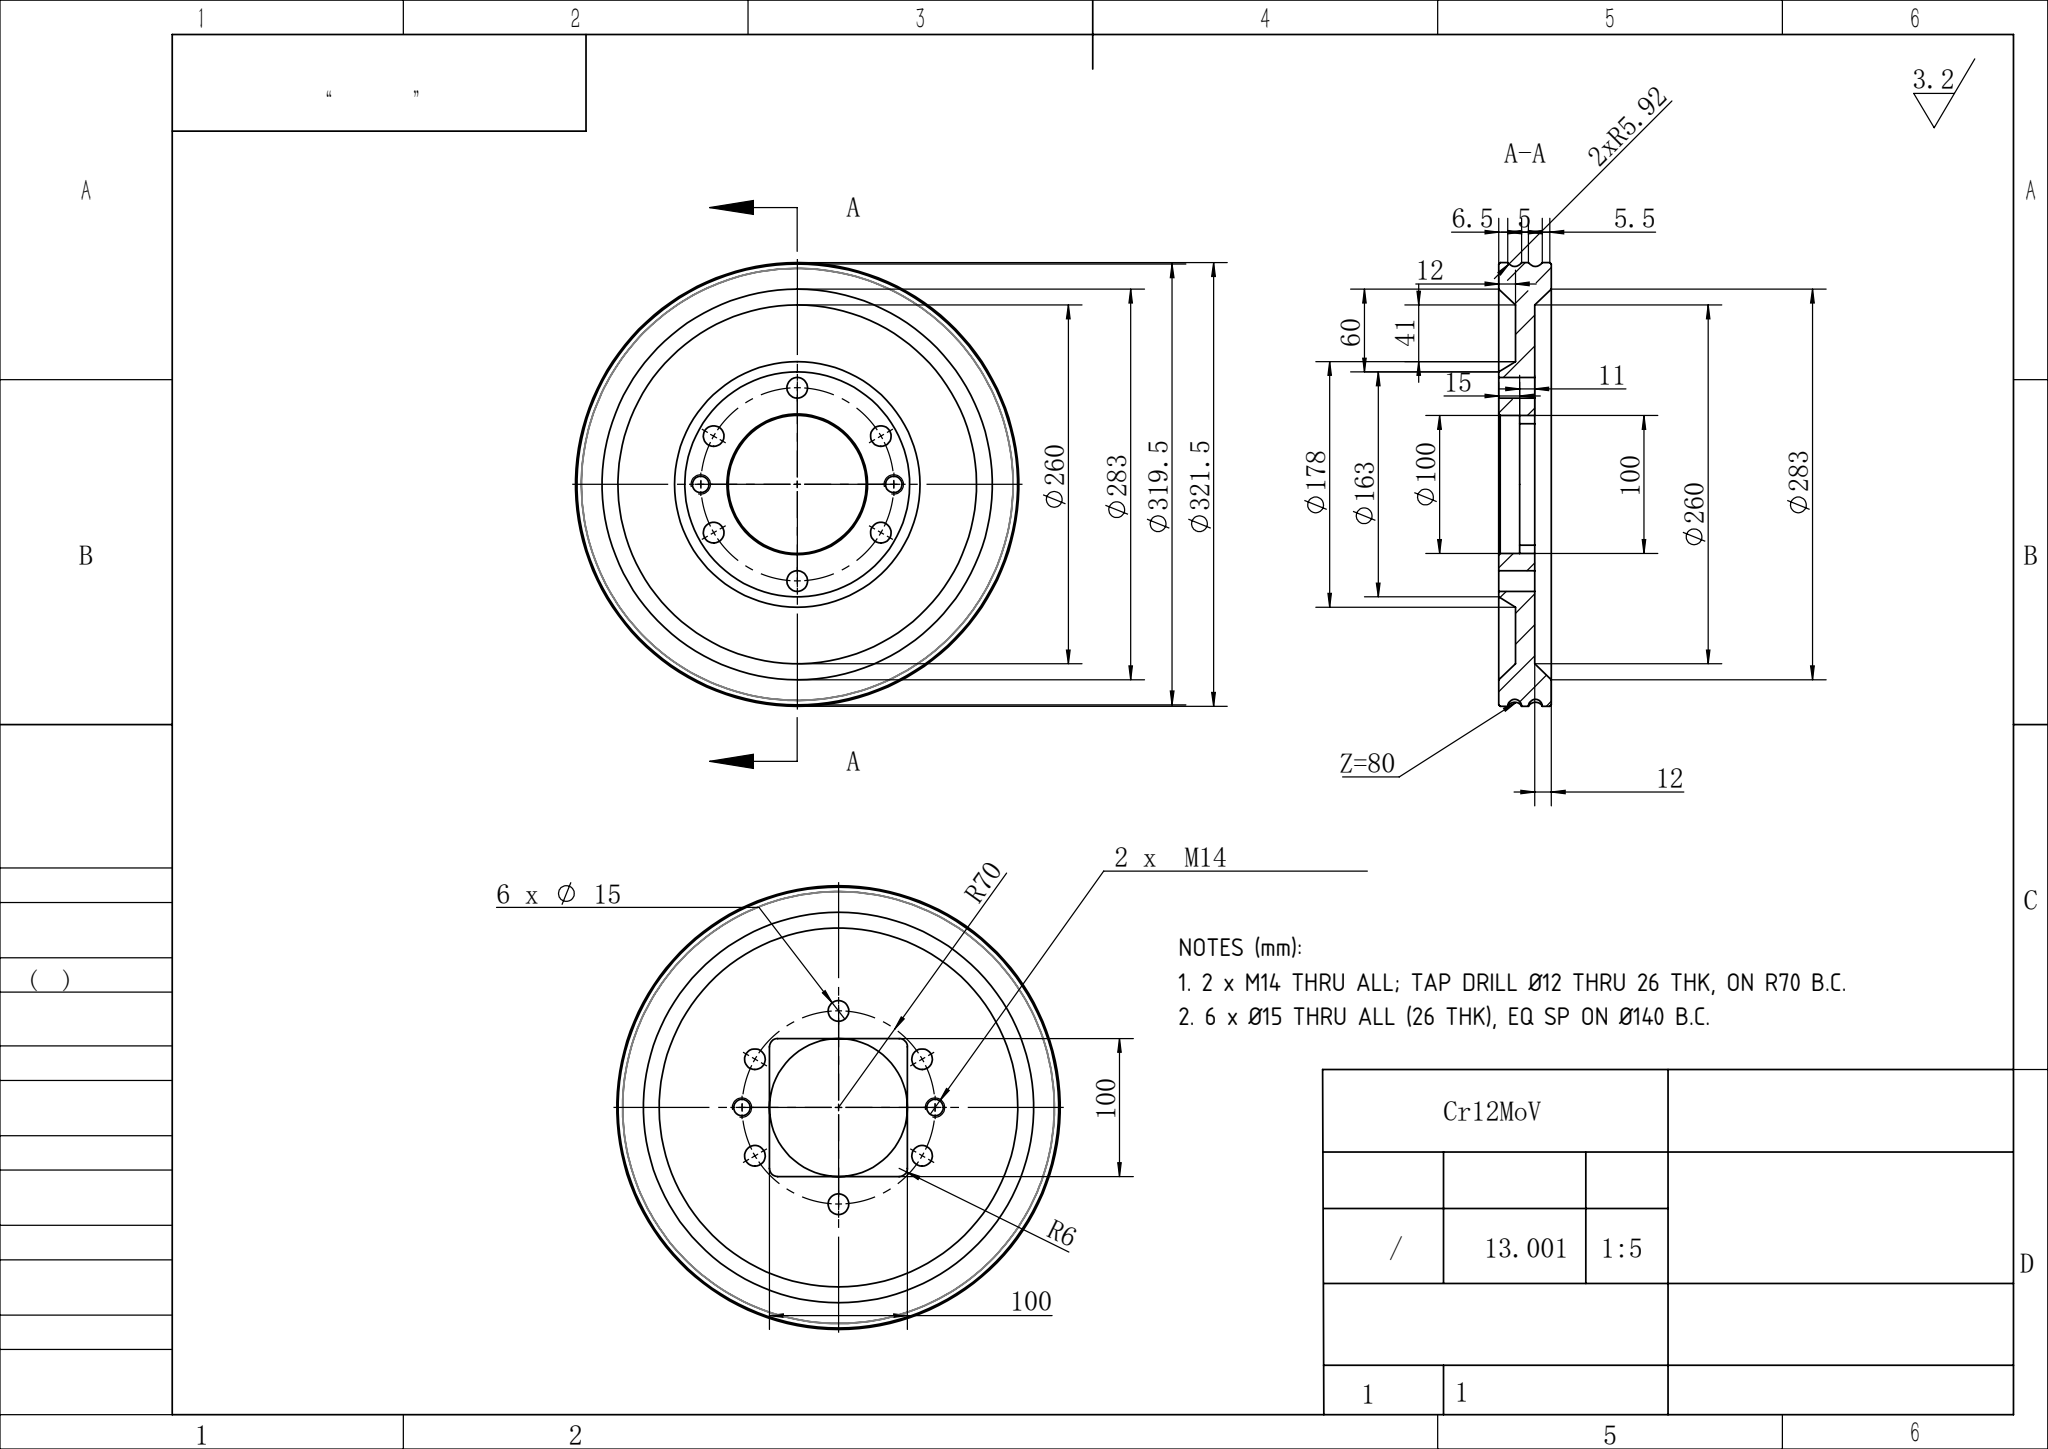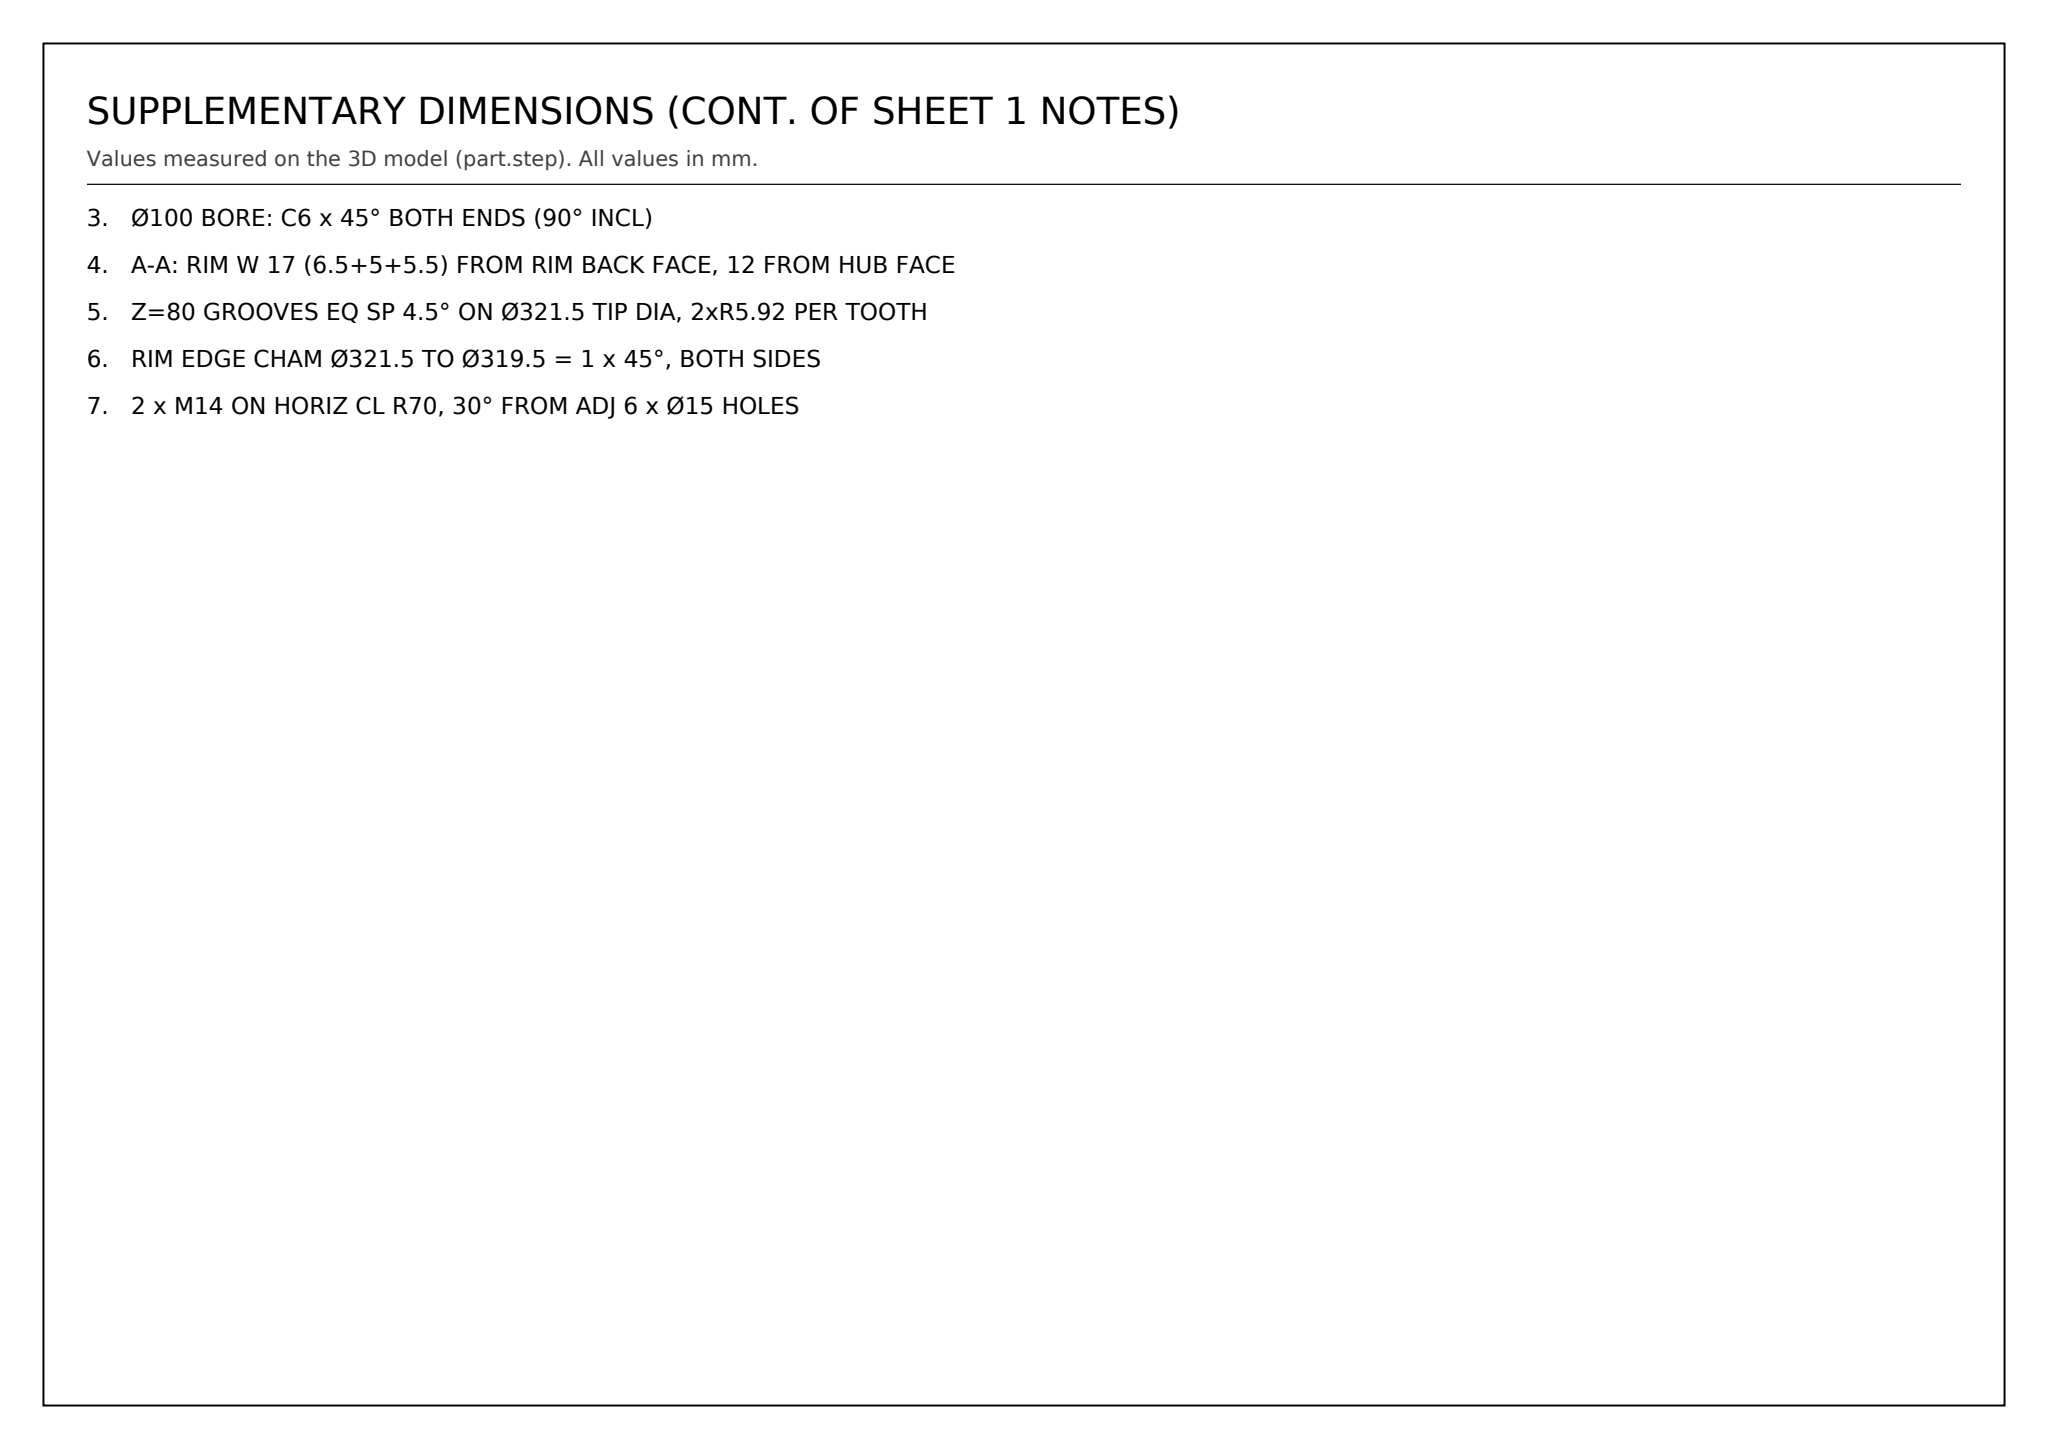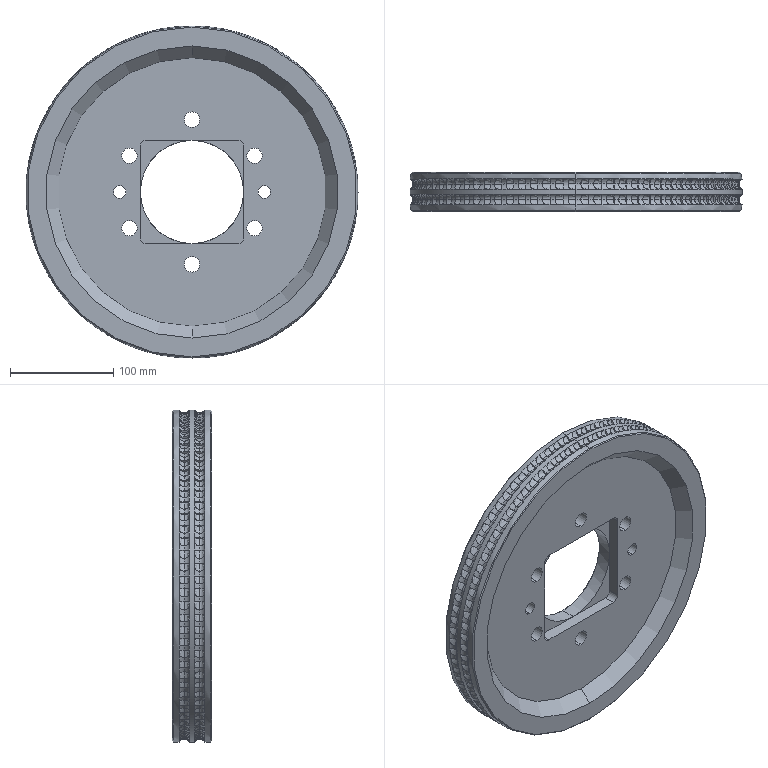Part | SolidWorks | mm | 1 solid | 851 faces | box 321.5 x 38 x 321.5 mm | volume 1656237 mm3 | spline 320 | torus 318 | plane 173 | cylinder 28 | cone 12 | commonest cylinder face diameters 15 x12 12 x8 321.5 x6 100 x2
Drawing notes:
2 x M14 THRU ALL; TAP DRILL Ø12 THRU 26 THK, ON R70 B.C. | from the solid: cylinders [12.0,'y',[666.85,null,736.85],26.0] and [12.0,'y',[806.85,null,736.85],26.0] = ±70 from axis at 736.85, full 26 hub thk (y=12..38)
6 x Ø15 THRU ALL (26 THK), EQ SP ON Ø140 B.C. | from the solid: six Ø15 y-axis cylinders, L=26, centers at radius sqrt(60.62^2+35^2)=70 from (736.85,736.85)
Ø100 BORE: C6 x 45° BOTH ENDS (90° INCL) | from the solid: cones [90.0 incl, ref dia 100, count 2]; bore Ø100 L=14 within 26 thk hub -> (26-14)/2 = 6 axial = 6 radial at 45°
A-A: RIM W 17 (6.5+5+5.5) FROM RIM BACK FACE, 12 FROM HUB FACE | from the solid: Ø321.5 lands L=5 and L=5.5 with 6.5 lead-in = 17 rim width; y planes 0 (rim face) and 12 (hub face), bbox y=38
Z=80 GROOVES EQ SP 4.5° ON Ø321.5 TIP DIA, 2xR5.92 PER TOOTH | from the solid: Ø321.5 cyl (y-axis) + fillet_radii 5.92 (318 faces) ≈ 4 arcs x 80 teeth; 360/80=4.5°
RIM EDGE CHAM Ø321.5 TO Ø319.5 = 1 x 45°, BOTH SIDES | from the solid: cones 90° incl at ref_dia 321.5 and 319.5 (2 ea): radial 1.0 -> axial 1.0 at 45°
2 x M14 ON HORIZ CL R70, 30° FROM ADJ 6 x Ø15 HOLES | from the solid: Ø12 thru holes at (666.85,736.85)&(806.85,736.85)=R70 on X axis; Ø15 holes at R70 every 60° starting on Z axis (736.85,666.85)